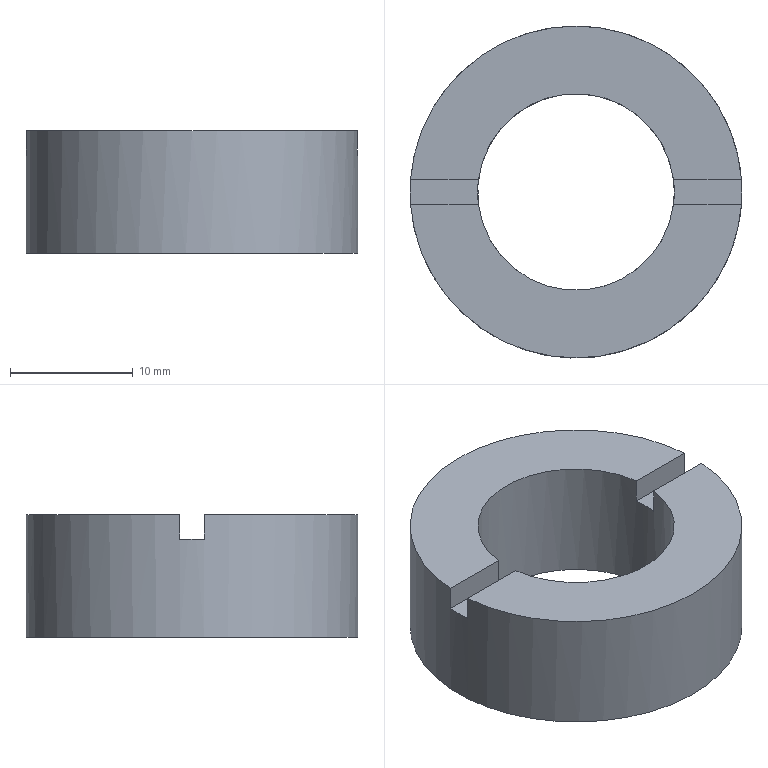Component | NX | GLAND | 1 solid | 11 faces | box 27 x 27 x 10 mm | volume 3671 mm3 | plane 9 | cylinder 2 | commonest cylinder face diameters 27 x1 16 x1
STEP:
#1=CARTESIAN_POINT('',(0.,0.,0.));
#2=DIRECTION('',(0.,0.,1.));
#3=DIRECTION('',(1.,0.,0.));
#4=AXIS2_PLACEMENT_3D('',#1,#2,#3);
#5=CARTESIAN_POINT('',(163.702,25.5,84.));
#6=VERTEX_POINT('',#5);
#7=CARTESIAN_POINT('',(169.228,25.5,84.));
#8=VERTEX_POINT('',#7);
#9=CARTESIAN_POINT('',(153.665,25.5,84.));
#10=DIRECTION('',(1.,0.,0.));
#11=VECTOR('',#10,1.);
#12=LINE('',#9,#11);
#13=CARTESIAN_POINT('',(177.165,26.5,84.));
#14=DIRECTION('',(0.,0.,1.));
#15=DIRECTION('',(1.,0.,0.));
#16=AXIS2_PLACEMENT_3D('',#13,#14,#15);
#17=PLANE('',#16);
#18=CARTESIAN_POINT('',(-23.5,-1.));
#19=DIRECTION('',(1.,0.));
#20=VECTOR('',#19,1.);
#21=LINE('',#18,#20);
#22=(GEOMETRIC_REPRESENTATION_CONTEXT(2)PARAMETRIC_REPRESENTATION_CONTEXT()REPRESENTATION_CONTEXT('',''));
#23=DEFINITIONAL_REPRESENTATION('',(#21),#22);
#24=PCURVE('',#17,#23);
#25=CARTESIAN_POINT('',(153.665,25.5,82.));
#26=DIRECTION('',(0.,-1.,0.));
#27=DIRECTION('',(0.,0.,-1.));
#28=AXIS2_PLACEMENT_3D('',#25,#26,#27);
#29=PLANE('',#28);
#30=CARTESIAN_POINT('',(-2.,0.));
#31=DIRECTION('',(0.,1.));
#32=VECTOR('',#31,1.);
#33=LINE('',#30,#32);
#34=(GEOMETRIC_REPRESENTATION_CONTEXT(2)PARAMETRIC_REPRESENTATION_CONTEXT()REPRESENTATION_CONTEXT('',''));
#35=DEFINITIONAL_REPRESENTATION('',(#33),#34);
#36=PCURVE('',#29,#35);
#37=SURFACE_CURVE('',#12,(#24,#36),.PCURVE_S1.);
#38=EDGE_CURVE('',#6,#8,#37,.T.);
#39=ORIENTED_EDGE('',*,*,#38,.F.);
#40=CARTESIAN_POINT('',(190.628,25.5,84.));
#41=VERTEX_POINT('',#40);
#42=CARTESIAN_POINT('',(177.165,26.5,84.));
#43=DIRECTION('',(0.,0.,1.));
#44=DIRECTION('',(1.,0.,0.));
#45=AXIS2_PLACEMENT_3D('',#42,#43,#44);
#46=CIRCLE('',#45,13.5);
#47=CARTESIAN_POINT('',(0.,0.));
#48=DIRECTION('',(1.,0.));
#49=AXIS2_PLACEMENT_2D('',#47,#48);
#50=CIRCLE('',#49,13.5);
#51=(GEOMETRIC_REPRESENTATION_CONTEXT(2)PARAMETRIC_REPRESENTATION_CONTEXT()REPRESENTATION_CONTEXT('',''));
#52=DEFINITIONAL_REPRESENTATION('',(#50),#51);
#53=PCURVE('',#17,#52);
#54=CARTESIAN_POINT('',(177.165,26.5,84.));
#55=DIRECTION('',(0.,0.,-1.));
#56=DIRECTION('',(-1.,0.,0.));
#57=AXIS2_PLACEMENT_3D('',#54,#55,#56);
#58=CYLINDRICAL_SURFACE('',#57,13.5);
#59=CARTESIAN_POINT('',(15.708,0.));
#60=DIRECTION('',(-1.,0.));
#61=VECTOR('',#60,1.);
#62=LINE('',#59,#61);
#63=(GEOMETRIC_REPRESENTATION_CONTEXT(2)PARAMETRIC_REPRESENTATION_CONTEXT()REPRESENTATION_CONTEXT('',''));
#64=DEFINITIONAL_REPRESENTATION('',(#62),#63);
#65=PCURVE('',#58,#64);
#66=SURFACE_CURVE('',#46,(#53,#65),.PCURVE_S1.);
#67=EDGE_CURVE('',#6,#41,#66,.T.);
#68=ORIENTED_EDGE('',*,*,#67,.T.);
#69=CARTESIAN_POINT('',(185.103,25.5,84.));
#70=VERTEX_POINT('',#69);
#71=CARTESIAN_POINT('',(153.665,25.5,84.));
#72=DIRECTION('',(1.,0.,0.));
#73=VECTOR('',#72,1.);
#74=LINE('',#71,#73);
#75=CARTESIAN_POINT('',(-23.5,-1.));
#76=DIRECTION('',(1.,0.));
#77=VECTOR('',#76,1.);
#78=LINE('',#75,#77);
#79=(GEOMETRIC_REPRESENTATION_CONTEXT(2)PARAMETRIC_REPRESENTATION_CONTEXT()REPRESENTATION_CONTEXT('',''));
#80=DEFINITIONAL_REPRESENTATION('',(#78),#79);
#81=PCURVE('',#17,#80);
#82=CARTESIAN_POINT('',(153.665,25.5,82.));
#83=DIRECTION('',(0.,-1.,0.));
#84=DIRECTION('',(0.,0.,-1.));
#85=AXIS2_PLACEMENT_3D('',#82,#83,#84);
#86=PLANE('',#85);
#87=CARTESIAN_POINT('',(-2.,0.));
#88=DIRECTION('',(0.,1.));
#89=VECTOR('',#88,1.);
#90=LINE('',#87,#89);
#91=(GEOMETRIC_REPRESENTATION_CONTEXT(2)PARAMETRIC_REPRESENTATION_CONTEXT()REPRESENTATION_CONTEXT('',''));
#92=DEFINITIONAL_REPRESENTATION('',(#90),#91);
#93=PCURVE('',#86,#92);
#94=SURFACE_CURVE('',#74,(#81,#93),.PCURVE_S1.);
#95=EDGE_CURVE('',#70,#41,#94,.T.);
#96=ORIENTED_EDGE('',*,*,#95,.F.);
#97=CARTESIAN_POINT('',(177.165,26.5,84.));
#98=DIRECTION('',(0.,0.,1.));
#99=DIRECTION('',(1.,0.,0.));
#100=AXIS2_PLACEMENT_3D('',#97,#98,#99);
#101=CIRCLE('',#100,8.);
#102=CARTESIAN_POINT('',(0.,0.));
#103=DIRECTION('',(1.,0.));
#104=AXIS2_PLACEMENT_2D('',#102,#103);
#105=CIRCLE('',#104,8.);
#106=(GEOMETRIC_REPRESENTATION_CONTEXT(2)PARAMETRIC_REPRESENTATION_CONTEXT()REPRESENTATION_CONTEXT('',''));
#107=DEFINITIONAL_REPRESENTATION('',(#105),#106);
#108=PCURVE('',#17,#107);
#109=CARTESIAN_POINT('',(177.165,26.5,84.));
#110=DIRECTION('',(0.,0.,-1.));
#111=DIRECTION('',(-1.,0.,0.));
#112=AXIS2_PLACEMENT_3D('',#109,#110,#111);
#113=CYLINDRICAL_SURFACE('',#112,8.);
#114=CARTESIAN_POINT('',(15.708,0.));
#115=DIRECTION('',(-1.,0.));
#116=VECTOR('',#115,1.);
#117=LINE('',#114,#116);
#118=(GEOMETRIC_REPRESENTATION_CONTEXT(2)PARAMETRIC_REPRESENTATION_CONTEXT()REPRESENTATION_CONTEXT('',''));
#119=DEFINITIONAL_REPRESENTATION('',(#117),#118);
#120=PCURVE('',#113,#119);
#121=SURFACE_CURVE('',#101,(#108,#120),.PCURVE_S1.);
#122=EDGE_CURVE('',#8,#70,#121,.T.);
#123=ORIENTED_EDGE('',*,*,#122,.F.);
#124=EDGE_LOOP('',(#39,#68,#96,#123));
#125=FACE_BOUND('',#124,.T.);
#126=ADVANCED_FACE('',(#125),#17,.T.);
#127=ORIENTED_EDGE('',*,*,#67,.F.);
#128=CARTESIAN_POINT('',(163.702,25.5,82.));
#129=VERTEX_POINT('',#128);
#130=CARTESIAN_POINT('',(163.702,25.5,84.));
#131=DIRECTION('',(0.,0.,-1.));
#132=VECTOR('',#131,1.);
#133=LINE('',#130,#132);
#134=CARTESIAN_POINT('',(12.492,0.));
#135=DIRECTION('',(0.,1.));
#136=VECTOR('',#135,1.);
#137=LINE('',#134,#136);
#138=(GEOMETRIC_REPRESENTATION_CONTEXT(2)PARAMETRIC_REPRESENTATION_CONTEXT()REPRESENTATION_CONTEXT('',''));
#139=DEFINITIONAL_REPRESENTATION('',(#137),#138);
#140=PCURVE('',#58,#139);
#141=CARTESIAN_POINT('',(-2.,10.037));
#142=DIRECTION('',(1.,0.));
#143=VECTOR('',#142,1.);
#144=LINE('',#141,#143);
#145=(GEOMETRIC_REPRESENTATION_CONTEXT(2)PARAMETRIC_REPRESENTATION_CONTEXT()REPRESENTATION_CONTEXT('',''));
#146=DEFINITIONAL_REPRESENTATION('',(#144),#145);
#147=PCURVE('',#29,#146);
#148=SURFACE_CURVE('',#133,(#140,#147),.PCURVE_S1.);
#149=EDGE_CURVE('',#6,#129,#148,.T.);
#150=ORIENTED_EDGE('',*,*,#149,.T.);
#151=CARTESIAN_POINT('',(163.702,25.5,74.));
#152=VERTEX_POINT('',#151);
#153=CARTESIAN_POINT('',(163.702,25.5,82.));
#154=CARTESIAN_POINT('',(163.702,25.5,74.));
#155=B_SPLINE_CURVE_WITH_KNOTS('',1,(#153,#154),.UNSPECIFIED.,.F.,.F.,(2,2),(2.,10.),.PIECEWISE_BEZIER_KNOTS.);
#156=CARTESIAN_POINT('',(12.492,0.));
#157=DIRECTION('',(0.,1.));
#158=VECTOR('',#157,1.);
#159=LINE('',#156,#158);
#160=(GEOMETRIC_REPRESENTATION_CONTEXT(2)PARAMETRIC_REPRESENTATION_CONTEXT()REPRESENTATION_CONTEXT('',''));
#161=DEFINITIONAL_REPRESENTATION('',(#159),#160);
#162=PCURVE('',#58,#161);
#163=CARTESIAN_POINT('',(6.209,0.));
#164=DIRECTION('',(0.,1.));
#165=VECTOR('',#164,1.);
#166=LINE('',#163,#165);
#167=(GEOMETRIC_REPRESENTATION_CONTEXT(2)PARAMETRIC_REPRESENTATION_CONTEXT()REPRESENTATION_CONTEXT('',''));
#168=DEFINITIONAL_REPRESENTATION('',(#166),#167);
#169=PCURVE('',#58,#168);
#170=SEAM_CURVE('',#155,(#162,#169),.PCURVE_S1.);
#171=EDGE_CURVE('',#129,#152,#170,.T.);
#172=ORIENTED_EDGE('',*,*,#171,.T.);
#173=CARTESIAN_POINT('',(190.665,26.5,74.));
#174=VERTEX_POINT('',#173);
#175=CARTESIAN_POINT('',(177.165,26.5,74.));
#176=DIRECTION('',(0.,0.,1.));
#177=DIRECTION('',(1.,0.,0.));
#178=AXIS2_PLACEMENT_3D('',#175,#176,#177);
#179=CIRCLE('',#178,13.5);
#180=CARTESIAN_POINT('',(15.708,10.));
#181=DIRECTION('',(-1.,0.));
#182=VECTOR('',#181,1.);
#183=LINE('',#180,#182);
#184=(GEOMETRIC_REPRESENTATION_CONTEXT(2)PARAMETRIC_REPRESENTATION_CONTEXT()REPRESENTATION_CONTEXT('',''));
#185=DEFINITIONAL_REPRESENTATION('',(#183),#184);
#186=PCURVE('',#58,#185);
#187=CARTESIAN_POINT('',(177.165,26.5,74.));
#188=DIRECTION('',(0.,0.,1.));
#189=DIRECTION('',(1.,0.,0.));
#190=AXIS2_PLACEMENT_3D('',#187,#188,#189);
#191=PLANE('',#190);
#192=CARTESIAN_POINT('',(0.,0.));
#193=DIRECTION('',(1.,0.));
#194=AXIS2_PLACEMENT_2D('',#192,#193);
#195=CIRCLE('',#194,13.5);
#196=(GEOMETRIC_REPRESENTATION_CONTEXT(2)PARAMETRIC_REPRESENTATION_CONTEXT()REPRESENTATION_CONTEXT('',''));
#197=DEFINITIONAL_REPRESENTATION('',(#195),#196);
#198=PCURVE('',#191,#197);
#199=SURFACE_CURVE('',#179,(#186,#198),.PCURVE_S1.);
#200=EDGE_CURVE('',#152,#174,#199,.T.);
#201=ORIENTED_EDGE('',*,*,#200,.T.);
#202=CARTESIAN_POINT('',(177.165,26.5,74.));
#203=DIRECTION('',(0.,0.,1.));
#204=DIRECTION('',(1.,0.,0.));
#205=AXIS2_PLACEMENT_3D('',#202,#203,#204);
#206=CIRCLE('',#205,13.5);
#207=CARTESIAN_POINT('',(9.425,10.));
#208=DIRECTION('',(-1.,0.));
#209=VECTOR('',#208,1.);
#210=LINE('',#207,#209);
#211=(GEOMETRIC_REPRESENTATION_CONTEXT(2)PARAMETRIC_REPRESENTATION_CONTEXT()REPRESENTATION_CONTEXT('',''));
#212=DEFINITIONAL_REPRESENTATION('',(#210),#211);
#213=PCURVE('',#58,#212);
#214=CARTESIAN_POINT('',(0.,0.));
#215=DIRECTION('',(1.,0.));
#216=AXIS2_PLACEMENT_2D('',#214,#215);
#217=CIRCLE('',#216,13.5);
#218=(GEOMETRIC_REPRESENTATION_CONTEXT(2)PARAMETRIC_REPRESENTATION_CONTEXT()REPRESENTATION_CONTEXT('',''));
#219=DEFINITIONAL_REPRESENTATION('',(#217),#218);
#220=PCURVE('',#191,#219);
#221=SURFACE_CURVE('',#206,(#213,#220),.PCURVE_S1.);
#222=EDGE_CURVE('',#174,#152,#221,.T.);
#223=ORIENTED_EDGE('',*,*,#222,.T.);
#224=ORIENTED_EDGE('',*,*,#171,.F.);
#225=CARTESIAN_POINT('',(163.702,27.5,82.));
#226=VERTEX_POINT('',#225);
#227=CARTESIAN_POINT('',(177.165,26.5,82.));
#228=DIRECTION('',(0.,0.,1.));
#229=DIRECTION('',(1.,0.,0.));
#230=AXIS2_PLACEMENT_3D('',#227,#228,#229);
#231=CIRCLE('',#230,13.5);
#232=CARTESIAN_POINT('',(9.425,2.));
#233=DIRECTION('',(-1.,0.));
#234=VECTOR('',#233,1.);
#235=LINE('',#232,#234);
#236=(GEOMETRIC_REPRESENTATION_CONTEXT(2)PARAMETRIC_REPRESENTATION_CONTEXT()REPRESENTATION_CONTEXT('',''));
#237=DEFINITIONAL_REPRESENTATION('',(#235),#236);
#238=PCURVE('',#58,#237);
#239=CARTESIAN_POINT('',(177.165,26.5,82.));
#240=DIRECTION('',(0.,0.,1.));
#241=DIRECTION('',(1.,0.,0.));
#242=AXIS2_PLACEMENT_3D('',#239,#240,#241);
#243=PLANE('',#242);
#244=CARTESIAN_POINT('',(0.,0.));
#245=DIRECTION('',(1.,0.));
#246=AXIS2_PLACEMENT_2D('',#244,#245);
#247=CIRCLE('',#246,13.5);
#248=(GEOMETRIC_REPRESENTATION_CONTEXT(2)PARAMETRIC_REPRESENTATION_CONTEXT()REPRESENTATION_CONTEXT('',''));
#249=DEFINITIONAL_REPRESENTATION('',(#247),#248);
#250=PCURVE('',#243,#249);
#251=SURFACE_CURVE('',#231,(#238,#250),.PCURVE_S1.);
#252=EDGE_CURVE('',#226,#129,#251,.T.);
#253=ORIENTED_EDGE('',*,*,#252,.F.);
#254=CARTESIAN_POINT('',(163.702,27.5,84.));
#255=VERTEX_POINT('',#254);
#256=CARTESIAN_POINT('',(163.702,27.5,84.));
#257=DIRECTION('',(0.,0.,1.));
#258=VECTOR('',#257,1.);
#259=LINE('',#256,#258);
#260=CARTESIAN_POINT('',(6.357,0.));
#261=DIRECTION('',(0.,-1.));
#262=VECTOR('',#261,1.);
#263=LINE('',#260,#262);
#264=(GEOMETRIC_REPRESENTATION_CONTEXT(2)PARAMETRIC_REPRESENTATION_CONTEXT()REPRESENTATION_CONTEXT('',''));
#265=DEFINITIONAL_REPRESENTATION('',(#263),#264);
#266=PCURVE('',#58,#265);
#267=CARTESIAN_POINT('',(200.665,27.5,82.));
#268=DIRECTION('',(0.,1.,0.));
#269=DIRECTION('',(0.,0.,1.));
#270=AXIS2_PLACEMENT_3D('',#267,#268,#269);
#271=PLANE('',#270);
#272=CARTESIAN_POINT('',(2.,-36.963));
#273=DIRECTION('',(1.,0.));
#274=VECTOR('',#273,1.);
#275=LINE('',#272,#274);
#276=(GEOMETRIC_REPRESENTATION_CONTEXT(2)PARAMETRIC_REPRESENTATION_CONTEXT()REPRESENTATION_CONTEXT('',''));
#277=DEFINITIONAL_REPRESENTATION('',(#275),#276);
#278=PCURVE('',#271,#277);
#279=SURFACE_CURVE('',#259,(#266,#278),.PCURVE_S1.);
#280=EDGE_CURVE('',#226,#255,#279,.T.);
#281=ORIENTED_EDGE('',*,*,#280,.T.);
#282=CARTESIAN_POINT('',(190.628,27.5,84.));
#283=VERTEX_POINT('',#282);
#284=CARTESIAN_POINT('',(177.165,26.5,84.));
#285=DIRECTION('',(0.,0.,1.));
#286=DIRECTION('',(1.,0.,0.));
#287=AXIS2_PLACEMENT_3D('',#284,#285,#286);
#288=CIRCLE('',#287,13.5);
#289=CARTESIAN_POINT('',(9.425,0.));
#290=DIRECTION('',(-1.,0.));
#291=VECTOR('',#290,1.);
#292=LINE('',#289,#291);
#293=(GEOMETRIC_REPRESENTATION_CONTEXT(2)PARAMETRIC_REPRESENTATION_CONTEXT()REPRESENTATION_CONTEXT('',''));
#294=DEFINITIONAL_REPRESENTATION('',(#292),#293);
#295=PCURVE('',#58,#294);
#296=CARTESIAN_POINT('',(177.165,26.5,84.));
#297=DIRECTION('',(0.,0.,1.));
#298=DIRECTION('',(1.,0.,0.));
#299=AXIS2_PLACEMENT_3D('',#296,#297,#298);
#300=PLANE('',#299);
#301=CARTESIAN_POINT('',(0.,0.));
#302=DIRECTION('',(1.,0.));
#303=AXIS2_PLACEMENT_2D('',#301,#302);
#304=CIRCLE('',#303,13.5);
#305=(GEOMETRIC_REPRESENTATION_CONTEXT(2)PARAMETRIC_REPRESENTATION_CONTEXT()REPRESENTATION_CONTEXT('',''));
#306=DEFINITIONAL_REPRESENTATION('',(#304),#305);
#307=PCURVE('',#300,#306);
#308=SURFACE_CURVE('',#288,(#295,#307),.PCURVE_S1.);
#309=EDGE_CURVE('',#283,#255,#308,.T.);
#310=ORIENTED_EDGE('',*,*,#309,.F.);
#311=CARTESIAN_POINT('',(190.628,27.5,82.));
#312=VERTEX_POINT('',#311);
#313=CARTESIAN_POINT('',(190.628,27.5,84.));
#314=DIRECTION('',(0.,0.,-1.));
#315=VECTOR('',#314,1.);
#316=LINE('',#313,#315);
#317=CARTESIAN_POINT('',(9.351,0.));
#318=DIRECTION('',(0.,1.));
#319=VECTOR('',#318,1.);
#320=LINE('',#317,#319);
#321=(GEOMETRIC_REPRESENTATION_CONTEXT(2)PARAMETRIC_REPRESENTATION_CONTEXT()REPRESENTATION_CONTEXT('',''));
#322=DEFINITIONAL_REPRESENTATION('',(#320),#321);
#323=PCURVE('',#58,#322);
#324=CARTESIAN_POINT('',(200.665,27.5,82.));
#325=DIRECTION('',(0.,1.,0.));
#326=DIRECTION('',(0.,0.,1.));
#327=AXIS2_PLACEMENT_3D('',#324,#325,#326);
#328=PLANE('',#327);
#329=CARTESIAN_POINT('',(2.,-10.037));
#330=DIRECTION('',(-1.,0.));
#331=VECTOR('',#330,1.);
#332=LINE('',#329,#331);
#333=(GEOMETRIC_REPRESENTATION_CONTEXT(2)PARAMETRIC_REPRESENTATION_CONTEXT()REPRESENTATION_CONTEXT('',''));
#334=DEFINITIONAL_REPRESENTATION('',(#332),#333);
#335=PCURVE('',#328,#334);
#336=SURFACE_CURVE('',#316,(#323,#335),.PCURVE_S1.);
#337=EDGE_CURVE('',#283,#312,#336,.T.);
#338=ORIENTED_EDGE('',*,*,#337,.T.);
#339=CARTESIAN_POINT('',(190.628,25.5,82.));
#340=VERTEX_POINT('',#339);
#341=CARTESIAN_POINT('',(177.165,26.5,82.));
#342=DIRECTION('',(0.,0.,1.));
#343=DIRECTION('',(1.,0.,0.));
#344=AXIS2_PLACEMENT_3D('',#341,#342,#343);
#345=CIRCLE('',#344,13.5);
#346=CARTESIAN_POINT('',(15.708,2.));
#347=DIRECTION('',(-1.,0.));
#348=VECTOR('',#347,1.);
#349=LINE('',#346,#348);
#350=(GEOMETRIC_REPRESENTATION_CONTEXT(2)PARAMETRIC_REPRESENTATION_CONTEXT()REPRESENTATION_CONTEXT('',''));
#351=DEFINITIONAL_REPRESENTATION('',(#349),#350);
#352=PCURVE('',#58,#351);
#353=CARTESIAN_POINT('',(177.165,26.5,82.));
#354=DIRECTION('',(0.,0.,1.));
#355=DIRECTION('',(1.,0.,0.));
#356=AXIS2_PLACEMENT_3D('',#353,#354,#355);
#357=PLANE('',#356);
#358=CARTESIAN_POINT('',(0.,0.));
#359=DIRECTION('',(1.,0.));
#360=AXIS2_PLACEMENT_2D('',#358,#359);
#361=CIRCLE('',#360,13.5);
#362=(GEOMETRIC_REPRESENTATION_CONTEXT(2)PARAMETRIC_REPRESENTATION_CONTEXT()REPRESENTATION_CONTEXT('',''));
#363=DEFINITIONAL_REPRESENTATION('',(#361),#362);
#364=PCURVE('',#357,#363);
#365=SURFACE_CURVE('',#345,(#352,#364),.PCURVE_S1.);
#366=EDGE_CURVE('',#340,#312,#365,.T.);
#367=ORIENTED_EDGE('',*,*,#366,.F.);
#368=CARTESIAN_POINT('',(190.628,25.5,84.));
#369=DIRECTION('',(0.,0.,1.));
#370=VECTOR('',#369,1.);
#371=LINE('',#368,#370);
#372=CARTESIAN_POINT('',(9.499,0.));
#373=DIRECTION('',(0.,-1.));
#374=VECTOR('',#373,1.);
#375=LINE('',#372,#374);
#376=(GEOMETRIC_REPRESENTATION_CONTEXT(2)PARAMETRIC_REPRESENTATION_CONTEXT()REPRESENTATION_CONTEXT('',''));
#377=DEFINITIONAL_REPRESENTATION('',(#375),#376);
#378=PCURVE('',#58,#377);
#379=CARTESIAN_POINT('',(-2.,36.963));
#380=DIRECTION('',(-1.,0.));
#381=VECTOR('',#380,1.);
#382=LINE('',#379,#381);
#383=(GEOMETRIC_REPRESENTATION_CONTEXT(2)PARAMETRIC_REPRESENTATION_CONTEXT()REPRESENTATION_CONTEXT('',''));
#384=DEFINITIONAL_REPRESENTATION('',(#382),#383);
#385=PCURVE('',#86,#384);
#386=SURFACE_CURVE('',#371,(#378,#385),.PCURVE_S1.);
#387=EDGE_CURVE('',#340,#41,#386,.T.);
#388=ORIENTED_EDGE('',*,*,#387,.T.);
#389=EDGE_LOOP('',(#127,#150,#172,#201,#223,#224,#253,#281,#310,#338,#367,#388));
#390=FACE_BOUND('',#389,.T.);
#391=ADVANCED_FACE('',(#390),#58,.T.);
#392=CARTESIAN_POINT('',(169.228,27.5,82.));
#393=VERTEX_POINT('',#392);
#394=CARTESIAN_POINT('',(169.228,25.5,82.));
#395=VERTEX_POINT('',#394);
#396=CARTESIAN_POINT('',(177.165,26.5,82.));
#397=DIRECTION('',(0.,0.,1.));
#398=DIRECTION('',(1.,0.,0.));
#399=AXIS2_PLACEMENT_3D('',#396,#397,#398);
#400=CIRCLE('',#399,8.);
#401=CARTESIAN_POINT('',(9.425,2.));
#402=DIRECTION('',(-1.,0.));
#403=VECTOR('',#402,1.);
#404=LINE('',#401,#403);
#405=(GEOMETRIC_REPRESENTATION_CONTEXT(2)PARAMETRIC_REPRESENTATION_CONTEXT()REPRESENTATION_CONTEXT('',''));
#406=DEFINITIONAL_REPRESENTATION('',(#404),#405);
#407=PCURVE('',#113,#406);
#408=CARTESIAN_POINT('',(0.,0.));
#409=DIRECTION('',(1.,0.));
#410=AXIS2_PLACEMENT_2D('',#408,#409);
#411=CIRCLE('',#410,8.);
#412=(GEOMETRIC_REPRESENTATION_CONTEXT(2)PARAMETRIC_REPRESENTATION_CONTEXT()REPRESENTATION_CONTEXT('',''));
#413=DEFINITIONAL_REPRESENTATION('',(#411),#412);
#414=PCURVE('',#243,#413);
#415=SURFACE_CURVE('',#400,(#407,#414),.PCURVE_S1.);
#416=EDGE_CURVE('',#393,#395,#415,.T.);
#417=ORIENTED_EDGE('',*,*,#416,.F.);
#418=CARTESIAN_POINT('',(169.228,27.5,84.));
#419=VERTEX_POINT('',#418);
#420=CARTESIAN_POINT('',(169.228,27.5,84.));
#421=DIRECTION('',(0.,0.,1.));
#422=VECTOR('',#421,1.);
#423=LINE('',#420,#422);
#424=CARTESIAN_POINT('',(6.409,0.));
#425=DIRECTION('',(0.,-1.));
#426=VECTOR('',#425,1.);
#427=LINE('',#424,#426);
#428=(GEOMETRIC_REPRESENTATION_CONTEXT(2)PARAMETRIC_REPRESENTATION_CONTEXT()REPRESENTATION_CONTEXT('',''));
#429=DEFINITIONAL_REPRESENTATION('',(#427),#428);
#430=PCURVE('',#113,#429);
#431=CARTESIAN_POINT('',(2.,-31.437));
#432=DIRECTION('',(1.,0.));
#433=VECTOR('',#432,1.);
#434=LINE('',#431,#433);
#435=(GEOMETRIC_REPRESENTATION_CONTEXT(2)PARAMETRIC_REPRESENTATION_CONTEXT()REPRESENTATION_CONTEXT('',''));
#436=DEFINITIONAL_REPRESENTATION('',(#434),#435);
#437=PCURVE('',#271,#436);
#438=SURFACE_CURVE('',#423,(#430,#437),.PCURVE_S1.);
#439=EDGE_CURVE('',#393,#419,#438,.T.);
#440=ORIENTED_EDGE('',*,*,#439,.T.);
#441=CARTESIAN_POINT('',(185.103,27.5,84.));
#442=VERTEX_POINT('',#441);
#443=CARTESIAN_POINT('',(177.165,26.5,84.));
#444=DIRECTION('',(0.,0.,1.));
#445=DIRECTION('',(1.,0.,0.));
#446=AXIS2_PLACEMENT_3D('',#443,#444,#445);
#447=CIRCLE('',#446,8.);
#448=CARTESIAN_POINT('',(9.425,0.));
#449=DIRECTION('',(-1.,0.));
#450=VECTOR('',#449,1.);
#451=LINE('',#448,#450);
#452=(GEOMETRIC_REPRESENTATION_CONTEXT(2)PARAMETRIC_REPRESENTATION_CONTEXT()REPRESENTATION_CONTEXT('',''));
#453=DEFINITIONAL_REPRESENTATION('',(#451),#452);
#454=PCURVE('',#113,#453);
#455=CARTESIAN_POINT('',(0.,0.));
#456=DIRECTION('',(1.,0.));
#457=AXIS2_PLACEMENT_2D('',#455,#456);
#458=CIRCLE('',#457,8.);
#459=(GEOMETRIC_REPRESENTATION_CONTEXT(2)PARAMETRIC_REPRESENTATION_CONTEXT()REPRESENTATION_CONTEXT('',''));
#460=DEFINITIONAL_REPRESENTATION('',(#458),#459);
#461=PCURVE('',#300,#460);
#462=SURFACE_CURVE('',#447,(#454,#461),.PCURVE_S1.);
#463=EDGE_CURVE('',#442,#419,#462,.T.);
#464=ORIENTED_EDGE('',*,*,#463,.F.);
#465=CARTESIAN_POINT('',(185.103,27.5,82.));
#466=VERTEX_POINT('',#465);
#467=CARTESIAN_POINT('',(185.103,27.5,84.));
#468=DIRECTION('',(0.,0.,-1.));
#469=VECTOR('',#468,1.);
#470=LINE('',#467,#469);
#471=CARTESIAN_POINT('',(9.299,0.));
#472=DIRECTION('',(0.,1.));
#473=VECTOR('',#472,1.);
#474=LINE('',#471,#473);
#475=(GEOMETRIC_REPRESENTATION_CONTEXT(2)PARAMETRIC_REPRESENTATION_CONTEXT()REPRESENTATION_CONTEXT('',''));
#476=DEFINITIONAL_REPRESENTATION('',(#474),#475);
#477=PCURVE('',#113,#476);
#478=CARTESIAN_POINT('',(2.,-15.563));
#479=DIRECTION('',(-1.,0.));
#480=VECTOR('',#479,1.);
#481=LINE('',#478,#480);
#482=(GEOMETRIC_REPRESENTATION_CONTEXT(2)PARAMETRIC_REPRESENTATION_CONTEXT()REPRESENTATION_CONTEXT('',''));
#483=DEFINITIONAL_REPRESENTATION('',(#481),#482);
#484=PCURVE('',#328,#483);
#485=SURFACE_CURVE('',#470,(#477,#484),.PCURVE_S1.);
#486=EDGE_CURVE('',#442,#466,#485,.T.);
#487=ORIENTED_EDGE('',*,*,#486,.T.);
#488=CARTESIAN_POINT('',(185.103,25.5,82.));
#489=VERTEX_POINT('',#488);
#490=CARTESIAN_POINT('',(177.165,26.5,82.));
#491=DIRECTION('',(0.,0.,1.));
#492=DIRECTION('',(1.,0.,0.));
#493=AXIS2_PLACEMENT_3D('',#490,#491,#492);
#494=CIRCLE('',#493,8.);
#495=CARTESIAN_POINT('',(15.708,2.));
#496=DIRECTION('',(-1.,0.));
#497=VECTOR('',#496,1.);
#498=LINE('',#495,#497);
#499=(GEOMETRIC_REPRESENTATION_CONTEXT(2)PARAMETRIC_REPRESENTATION_CONTEXT()REPRESENTATION_CONTEXT('',''));
#500=DEFINITIONAL_REPRESENTATION('',(#498),#499);
#501=PCURVE('',#113,#500);
#502=CARTESIAN_POINT('',(0.,0.));
#503=DIRECTION('',(1.,0.));
#504=AXIS2_PLACEMENT_2D('',#502,#503);
#505=CIRCLE('',#504,8.);
#506=(GEOMETRIC_REPRESENTATION_CONTEXT(2)PARAMETRIC_REPRESENTATION_CONTEXT()REPRESENTATION_CONTEXT('',''));
#507=DEFINITIONAL_REPRESENTATION('',(#505),#506);
#508=PCURVE('',#357,#507);
#509=SURFACE_CURVE('',#494,(#501,#508),.PCURVE_S1.);
#510=EDGE_CURVE('',#489,#466,#509,.T.);
#511=ORIENTED_EDGE('',*,*,#510,.F.);
#512=CARTESIAN_POINT('',(185.103,25.5,84.));
#513=DIRECTION('',(0.,0.,1.));
#514=VECTOR('',#513,1.);
#515=LINE('',#512,#514);
#516=CARTESIAN_POINT('',(9.55,0.));
#517=DIRECTION('',(0.,-1.));
#518=VECTOR('',#517,1.);
#519=LINE('',#516,#518);
#520=(GEOMETRIC_REPRESENTATION_CONTEXT(2)PARAMETRIC_REPRESENTATION_CONTEXT()REPRESENTATION_CONTEXT('',''));
#521=DEFINITIONAL_REPRESENTATION('',(#519),#520);
#522=PCURVE('',#113,#521);
#523=CARTESIAN_POINT('',(-2.,31.437));
#524=DIRECTION('',(-1.,0.));
#525=VECTOR('',#524,1.);
#526=LINE('',#523,#525);
#527=(GEOMETRIC_REPRESENTATION_CONTEXT(2)PARAMETRIC_REPRESENTATION_CONTEXT()REPRESENTATION_CONTEXT('',''));
#528=DEFINITIONAL_REPRESENTATION('',(#526),#527);
#529=PCURVE('',#86,#528);
#530=SURFACE_CURVE('',#515,(#522,#529),.PCURVE_S1.);
#531=EDGE_CURVE('',#489,#70,#530,.T.);
#532=ORIENTED_EDGE('',*,*,#531,.T.);
#533=ORIENTED_EDGE('',*,*,#122,.F.);
#534=CARTESIAN_POINT('',(169.228,25.5,84.));
#535=DIRECTION('',(0.,0.,-1.));
#536=VECTOR('',#535,1.);
#537=LINE('',#534,#536);
#538=CARTESIAN_POINT('',(12.441,0.));
#539=DIRECTION('',(0.,1.));
#540=VECTOR('',#539,1.);
#541=LINE('',#538,#540);
#542=(GEOMETRIC_REPRESENTATION_CONTEXT(2)PARAMETRIC_REPRESENTATION_CONTEXT()REPRESENTATION_CONTEXT('',''));
#543=DEFINITIONAL_REPRESENTATION('',(#541),#542);
#544=PCURVE('',#113,#543);
#545=CARTESIAN_POINT('',(-2.,15.563));
#546=DIRECTION('',(1.,0.));
#547=VECTOR('',#546,1.);
#548=LINE('',#545,#547);
#549=(GEOMETRIC_REPRESENTATION_CONTEXT(2)PARAMETRIC_REPRESENTATION_CONTEXT()REPRESENTATION_CONTEXT('',''));
#550=DEFINITIONAL_REPRESENTATION('',(#548),#549);
#551=PCURVE('',#29,#550);
#552=SURFACE_CURVE('',#537,(#544,#551),.PCURVE_S1.);
#553=EDGE_CURVE('',#8,#395,#552,.T.);
#554=ORIENTED_EDGE('',*,*,#553,.T.);
#555=CARTESIAN_POINT('',(169.228,25.5,74.));
#556=VERTEX_POINT('',#555);
#557=CARTESIAN_POINT('',(169.228,25.5,82.));
#558=CARTESIAN_POINT('',(169.228,25.5,74.));
#559=B_SPLINE_CURVE_WITH_KNOTS('',1,(#557,#558),.UNSPECIFIED.,.F.,.F.,(2,2),(2.,10.),.PIECEWISE_BEZIER_KNOTS.);
#560=CARTESIAN_POINT('',(12.441,0.));
#561=DIRECTION('',(0.,1.));
#562=VECTOR('',#561,1.);
#563=LINE('',#560,#562);
#564=(GEOMETRIC_REPRESENTATION_CONTEXT(2)PARAMETRIC_REPRESENTATION_CONTEXT()REPRESENTATION_CONTEXT('',''));
#565=DEFINITIONAL_REPRESENTATION('',(#563),#564);
#566=PCURVE('',#113,#565);
#567=CARTESIAN_POINT('',(6.158,0.));
#568=DIRECTION('',(0.,1.));
#569=VECTOR('',#568,1.);
#570=LINE('',#567,#569);
#571=(GEOMETRIC_REPRESENTATION_CONTEXT(2)PARAMETRIC_REPRESENTATION_CONTEXT()REPRESENTATION_CONTEXT('',''));
#572=DEFINITIONAL_REPRESENTATION('',(#570),#571);
#573=PCURVE('',#113,#572);
#574=SEAM_CURVE('',#559,(#566,#573),.PCURVE_S1.);
#575=EDGE_CURVE('',#395,#556,#574,.T.);
#576=ORIENTED_EDGE('',*,*,#575,.T.);
#577=CARTESIAN_POINT('',(185.165,26.5,74.));
#578=VERTEX_POINT('',#577);
#579=CARTESIAN_POINT('',(177.165,26.5,74.));
#580=DIRECTION('',(0.,0.,1.));
#581=DIRECTION('',(1.,0.,0.));
#582=AXIS2_PLACEMENT_3D('',#579,#580,#581);
#583=CIRCLE('',#582,8.);
#584=CARTESIAN_POINT('',(15.708,10.));
#585=DIRECTION('',(-1.,0.));
#586=VECTOR('',#585,1.);
#587=LINE('',#584,#586);
#588=(GEOMETRIC_REPRESENTATION_CONTEXT(2)PARAMETRIC_REPRESENTATION_CONTEXT()REPRESENTATION_CONTEXT('',''));
#589=DEFINITIONAL_REPRESENTATION('',(#587),#588);
#590=PCURVE('',#113,#589);
#591=CARTESIAN_POINT('',(0.,0.));
#592=DIRECTION('',(1.,0.));
#593=AXIS2_PLACEMENT_2D('',#591,#592);
#594=CIRCLE('',#593,8.);
#595=(GEOMETRIC_REPRESENTATION_CONTEXT(2)PARAMETRIC_REPRESENTATION_CONTEXT()REPRESENTATION_CONTEXT('',''));
#596=DEFINITIONAL_REPRESENTATION('',(#594),#595);
#597=PCURVE('',#191,#596);
#598=SURFACE_CURVE('',#583,(#590,#597),.PCURVE_S1.);
#599=EDGE_CURVE('',#556,#578,#598,.T.);
#600=ORIENTED_EDGE('',*,*,#599,.T.);
#601=CARTESIAN_POINT('',(177.165,26.5,74.));
#602=DIRECTION('',(0.,0.,1.));
#603=DIRECTION('',(1.,0.,0.));
#604=AXIS2_PLACEMENT_3D('',#601,#602,#603);
#605=CIRCLE('',#604,8.);
#606=CARTESIAN_POINT('',(9.425,10.));
#607=DIRECTION('',(-1.,0.));
#608=VECTOR('',#607,1.);
#609=LINE('',#606,#608);
#610=(GEOMETRIC_REPRESENTATION_CONTEXT(2)PARAMETRIC_REPRESENTATION_CONTEXT()REPRESENTATION_CONTEXT('',''));
#611=DEFINITIONAL_REPRESENTATION('',(#609),#610);
#612=PCURVE('',#113,#611);
#613=CARTESIAN_POINT('',(0.,0.));
#614=DIRECTION('',(1.,0.));
#615=AXIS2_PLACEMENT_2D('',#613,#614);
#616=CIRCLE('',#615,8.);
#617=(GEOMETRIC_REPRESENTATION_CONTEXT(2)PARAMETRIC_REPRESENTATION_CONTEXT()REPRESENTATION_CONTEXT('',''));
#618=DEFINITIONAL_REPRESENTATION('',(#616),#617);
#619=PCURVE('',#191,#618);
#620=SURFACE_CURVE('',#605,(#612,#619),.PCURVE_S1.);
#621=EDGE_CURVE('',#578,#556,#620,.T.);
#622=ORIENTED_EDGE('',*,*,#621,.T.);
#623=ORIENTED_EDGE('',*,*,#575,.F.);
#624=EDGE_LOOP('',(#417,#440,#464,#487,#511,#532,#533,#554,#576,#600,#622,#623));
#625=FACE_BOUND('',#624,.F.);
#626=ADVANCED_FACE('',(#625),#113,.F.);
#627=CARTESIAN_POINT('',(200.665,27.5,84.));
#628=DIRECTION('',(-1.,0.,0.));
#629=VECTOR('',#628,1.);
#630=LINE('',#627,#629);
#631=CARTESIAN_POINT('',(23.5,1.));
#632=DIRECTION('',(-1.,0.));
#633=VECTOR('',#632,1.);
#634=LINE('',#631,#633);
#635=(GEOMETRIC_REPRESENTATION_CONTEXT(2)PARAMETRIC_REPRESENTATION_CONTEXT()REPRESENTATION_CONTEXT('',''));
#636=DEFINITIONAL_REPRESENTATION('',(#634),#635);
#637=PCURVE('',#300,#636);
#638=CARTESIAN_POINT('',(2.,0.));
#639=DIRECTION('',(0.,-1.));
#640=VECTOR('',#639,1.);
#641=LINE('',#638,#640);
#642=(GEOMETRIC_REPRESENTATION_CONTEXT(2)PARAMETRIC_REPRESENTATION_CONTEXT()REPRESENTATION_CONTEXT('',''));
#643=DEFINITIONAL_REPRESENTATION('',(#641),#642);
#644=PCURVE('',#328,#643);
#645=SURFACE_CURVE('',#630,(#637,#644),.PCURVE_S1.);
#646=EDGE_CURVE('',#283,#442,#645,.T.);
#647=ORIENTED_EDGE('',*,*,#646,.F.);
#648=ORIENTED_EDGE('',*,*,#309,.T.);
#649=CARTESIAN_POINT('',(200.665,27.5,84.));
#650=DIRECTION('',(-1.,0.,0.));
#651=VECTOR('',#650,1.);
#652=LINE('',#649,#651);
#653=CARTESIAN_POINT('',(23.5,1.));
#654=DIRECTION('',(-1.,0.));
#655=VECTOR('',#654,1.);
#656=LINE('',#653,#655);
#657=(GEOMETRIC_REPRESENTATION_CONTEXT(2)PARAMETRIC_REPRESENTATION_CONTEXT()REPRESENTATION_CONTEXT('',''));
#658=DEFINITIONAL_REPRESENTATION('',(#656),#657);
#659=PCURVE('',#300,#658);
#660=CARTESIAN_POINT('',(2.,0.));
#661=DIRECTION('',(0.,-1.));
#662=VECTOR('',#661,1.);
#663=LINE('',#660,#662);
#664=(GEOMETRIC_REPRESENTATION_CONTEXT(2)PARAMETRIC_REPRESENTATION_CONTEXT()REPRESENTATION_CONTEXT('',''));
#665=DEFINITIONAL_REPRESENTATION('',(#663),#664);
#666=PCURVE('',#271,#665);
#667=SURFACE_CURVE('',#652,(#659,#666),.PCURVE_S1.);
#668=EDGE_CURVE('',#419,#255,#667,.T.);
#669=ORIENTED_EDGE('',*,*,#668,.F.);
#670=ORIENTED_EDGE('',*,*,#463,.F.);
#671=EDGE_LOOP('',(#647,#648,#669,#670));
#672=FACE_BOUND('',#671,.T.);
#673=ADVANCED_FACE('',(#672),#300,.T.);
#674=ORIENTED_EDGE('',*,*,#222,.F.);
#675=ORIENTED_EDGE('',*,*,#200,.F.);
#676=EDGE_LOOP('',(#674,#675));
#677=FACE_BOUND('',#676,.T.);
#678=ORIENTED_EDGE('',*,*,#621,.T.);
#679=ORIENTED_EDGE('',*,*,#599,.T.);
#680=EDGE_LOOP('',(#678,#679));
#681=FACE_BOUND('',#680,.T.);
#682=ADVANCED_FACE('',(#677,#681),#191,.F.);
#683=ORIENTED_EDGE('',*,*,#366,.T.);
#684=CARTESIAN_POINT('',(200.665,27.5,82.));
#685=DIRECTION('',(1.,0.,0.));
#686=VECTOR('',#685,1.);
#687=LINE('',#684,#686);
#688=CARTESIAN_POINT('',(23.5,1.));
#689=DIRECTION('',(1.,0.));
#690=VECTOR('',#689,1.);
#691=LINE('',#688,#690);
#692=(GEOMETRIC_REPRESENTATION_CONTEXT(2)PARAMETRIC_REPRESENTATION_CONTEXT()REPRESENTATION_CONTEXT('',''));
#693=DEFINITIONAL_REPRESENTATION('',(#691),#692);
#694=PCURVE('',#357,#693);
#695=CARTESIAN_POINT('',(0.,0.));
#696=DIRECTION('',(0.,1.));
#697=VECTOR('',#696,1.);
#698=LINE('',#695,#697);
#699=(GEOMETRIC_REPRESENTATION_CONTEXT(2)PARAMETRIC_REPRESENTATION_CONTEXT()REPRESENTATION_CONTEXT('',''));
#700=DEFINITIONAL_REPRESENTATION('',(#698),#699);
#701=PCURVE('',#328,#700);
#702=SURFACE_CURVE('',#687,(#694,#701),.PCURVE_S1.);
#703=EDGE_CURVE('',#466,#312,#702,.T.);
#704=ORIENTED_EDGE('',*,*,#703,.F.);
#705=ORIENTED_EDGE('',*,*,#510,.F.);
#706=CARTESIAN_POINT('',(153.665,25.5,82.));
#707=DIRECTION('',(-1.,0.,0.));
#708=VECTOR('',#707,1.);
#709=LINE('',#706,#708);
#710=CARTESIAN_POINT('',(-23.5,-1.));
#711=DIRECTION('',(-1.,0.));
#712=VECTOR('',#711,1.);
#713=LINE('',#710,#712);
#714=(GEOMETRIC_REPRESENTATION_CONTEXT(2)PARAMETRIC_REPRESENTATION_CONTEXT()REPRESENTATION_CONTEXT('',''));
#715=DEFINITIONAL_REPRESENTATION('',(#713),#714);
#716=PCURVE('',#357,#715);
#717=CARTESIAN_POINT('',(0.,0.));
#718=DIRECTION('',(0.,-1.));
#719=VECTOR('',#718,1.);
#720=LINE('',#717,#719);
#721=(GEOMETRIC_REPRESENTATION_CONTEXT(2)PARAMETRIC_REPRESENTATION_CONTEXT()REPRESENTATION_CONTEXT('',''));
#722=DEFINITIONAL_REPRESENTATION('',(#720),#721);
#723=PCURVE('',#86,#722);
#724=SURFACE_CURVE('',#709,(#716,#723),.PCURVE_S1.);
#725=EDGE_CURVE('',#340,#489,#724,.T.);
#726=ORIENTED_EDGE('',*,*,#725,.F.);
#727=EDGE_LOOP('',(#683,#704,#705,#726));
#728=FACE_BOUND('',#727,.T.);
#729=ADVANCED_FACE('',(#728),#357,.T.);
#730=ORIENTED_EDGE('',*,*,#646,.T.);
#731=ORIENTED_EDGE('',*,*,#486,.T.);
#732=ORIENTED_EDGE('',*,*,#703,.T.);
#733=ORIENTED_EDGE('',*,*,#337,.F.);
#734=EDGE_LOOP('',(#730,#731,#732,#733));
#735=FACE_BOUND('',#734,.T.);
#736=ADVANCED_FACE('',(#735),#328,.F.);
#737=ORIENTED_EDGE('',*,*,#725,.T.);
#738=ORIENTED_EDGE('',*,*,#531,.T.);
#739=ORIENTED_EDGE('',*,*,#95,.T.);
#740=ORIENTED_EDGE('',*,*,#387,.F.);
#741=EDGE_LOOP('',(#737,#738,#739,#740));
#742=FACE_BOUND('',#741,.T.);
#743=ADVANCED_FACE('',(#742),#86,.F.);
#744=ORIENTED_EDGE('',*,*,#252,.T.);
#745=CARTESIAN_POINT('',(153.665,25.5,82.));
#746=DIRECTION('',(-1.,0.,0.));
#747=VECTOR('',#746,1.);
#748=LINE('',#745,#747);
#749=CARTESIAN_POINT('',(-23.5,-1.));
#750=DIRECTION('',(-1.,0.));
#751=VECTOR('',#750,1.);
#752=LINE('',#749,#751);
#753=(GEOMETRIC_REPRESENTATION_CONTEXT(2)PARAMETRIC_REPRESENTATION_CONTEXT()REPRESENTATION_CONTEXT('',''));
#754=DEFINITIONAL_REPRESENTATION('',(#752),#753);
#755=PCURVE('',#243,#754);
#756=CARTESIAN_POINT('',(0.,0.));
#757=DIRECTION('',(0.,-1.));
#758=VECTOR('',#757,1.);
#759=LINE('',#756,#758);
#760=(GEOMETRIC_REPRESENTATION_CONTEXT(2)PARAMETRIC_REPRESENTATION_CONTEXT()REPRESENTATION_CONTEXT('',''));
#761=DEFINITIONAL_REPRESENTATION('',(#759),#760);
#762=PCURVE('',#29,#761);
#763=SURFACE_CURVE('',#748,(#755,#762),.PCURVE_S1.);
#764=EDGE_CURVE('',#395,#129,#763,.T.);
#765=ORIENTED_EDGE('',*,*,#764,.F.);
#766=ORIENTED_EDGE('',*,*,#416,.F.);
#767=CARTESIAN_POINT('',(200.665,27.5,82.));
#768=DIRECTION('',(1.,0.,0.));
#769=VECTOR('',#768,1.);
#770=LINE('',#767,#769);
#771=CARTESIAN_POINT('',(23.5,1.));
#772=DIRECTION('',(1.,0.));
#773=VECTOR('',#772,1.);
#774=LINE('',#771,#773);
#775=(GEOMETRIC_REPRESENTATION_CONTEXT(2)PARAMETRIC_REPRESENTATION_CONTEXT()REPRESENTATION_CONTEXT('',''));
#776=DEFINITIONAL_REPRESENTATION('',(#774),#775);
#777=PCURVE('',#243,#776);
#778=CARTESIAN_POINT('',(0.,0.));
#779=DIRECTION('',(0.,1.));
#780=VECTOR('',#779,1.);
#781=LINE('',#778,#780);
#782=(GEOMETRIC_REPRESENTATION_CONTEXT(2)PARAMETRIC_REPRESENTATION_CONTEXT()REPRESENTATION_CONTEXT('',''));
#783=DEFINITIONAL_REPRESENTATION('',(#781),#782);
#784=PCURVE('',#271,#783);
#785=SURFACE_CURVE('',#770,(#777,#784),.PCURVE_S1.);
#786=EDGE_CURVE('',#226,#393,#785,.T.);
#787=ORIENTED_EDGE('',*,*,#786,.F.);
#788=EDGE_LOOP('',(#744,#765,#766,#787));
#789=FACE_BOUND('',#788,.T.);
#790=ADVANCED_FACE('',(#789),#243,.T.);
#791=ORIENTED_EDGE('',*,*,#38,.T.);
#792=ORIENTED_EDGE('',*,*,#553,.T.);
#793=ORIENTED_EDGE('',*,*,#764,.T.);
#794=ORIENTED_EDGE('',*,*,#149,.F.);
#795=EDGE_LOOP('',(#791,#792,#793,#794));
#796=FACE_BOUND('',#795,.T.);
#797=ADVANCED_FACE('',(#796),#29,.F.);
#798=ORIENTED_EDGE('',*,*,#786,.T.);
#799=ORIENTED_EDGE('',*,*,#439,.T.);
#800=ORIENTED_EDGE('',*,*,#668,.T.);
#801=ORIENTED_EDGE('',*,*,#280,.F.);
#802=EDGE_LOOP('',(#798,#799,#800,#801));
#803=FACE_BOUND('',#802,.T.);
#804=ADVANCED_FACE('',(#803),#271,.F.);
#805=CLOSED_SHELL('',(#126,#391,#626,#673,#682,#729,#736,#743,#790,#797,#804));
#806=MANIFOLD_SOLID_BREP('',#805);
#807=(LENGTH_UNIT()NAMED_UNIT(*)SI_UNIT(.MILLI.,.METRE.));
#808=UNCERTAINTY_MEASURE_WITH_UNIT(LENGTH_MEASURE(0.000002),#807,'','');
#809=(NAMED_UNIT(*)PLANE_ANGLE_UNIT()SI_UNIT($,.RADIAN.));
#810=(NAMED_UNIT(*)SI_UNIT($,.STERADIAN.)SOLID_ANGLE_UNIT());
#811=(GEOMETRIC_REPRESENTATION_CONTEXT(3)GLOBAL_UNCERTAINTY_ASSIGNED_CONTEXT((#808))GLOBAL_UNIT_ASSIGNED_CONTEXT((#807,#809,#810))REPRESENTATION_CONTEXT('',''));
#812=ADVANCED_BREP_SHAPE_REPRESENTATION('',(#4,#806),#811);